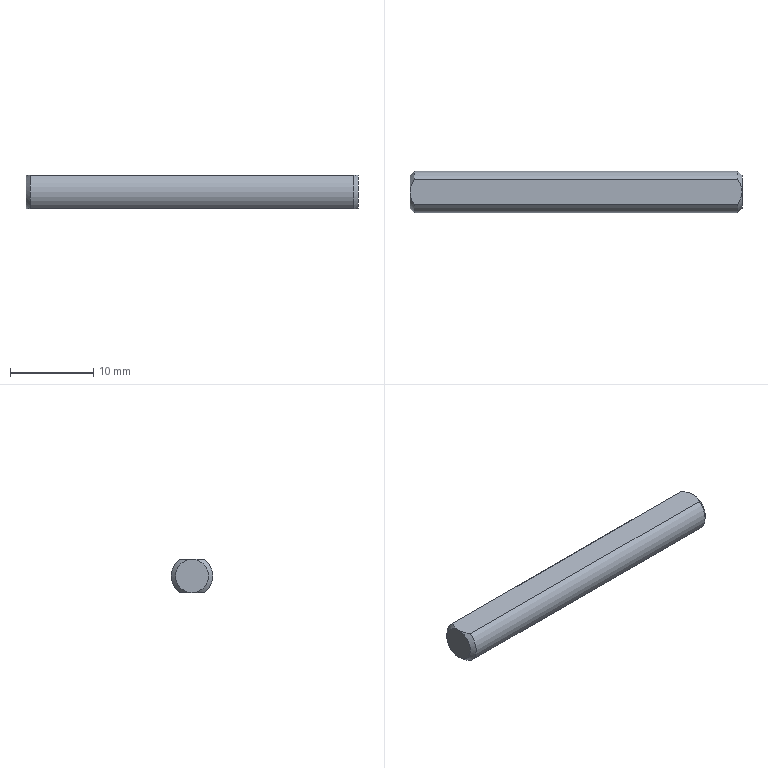Component | SolidWorks | 18ZTJ-NVT-01-003-1 | 1 solid | 10 faces | box 40 x 5 x 4 mm | volume 701 mm3 | cone 4 | plane 4 | cylinder 2 | commonest cylinder face diameters 5 x2 | material #45
build123d program:
from build123d import *

# Parameters (mm, degrees)
SKETCH1_R           = 2.5
BOSS_EXTRUDE1_DEPTH = 40
CHAMFER1_SIZE       = 0.5
CUT_EXTRUDE1_DEPTH  = 41.156


with BuildPart() as part:
    # Sketch1 → Boss-Extrude1 (new body)
    with BuildSketch(Plane(origin=(0, 0, 0), x_dir=(1, 0, 0), z_dir=(0, 1, 0))):
        with Locations(Location((0, 0, 0), (0, 0, 270))):
            Circle(SKETCH1_R)
    extrude(amount=BOSS_EXTRUDE1_DEPTH)

    # Chamfer1
    chamfer1_edges = [part.edges().sort_by_distance(p)[0] for p in [
        (0, 0, -2.5),
        (0, 40, -2.5),
    ]]
    chamfer(chamfer1_edges, length=CHAMFER1_SIZE)

    # Sketch2 → Cut-Extrude1 (cut, through all)
    with BuildSketch(Plane.XZ):
        with BuildLine():
            Line((-1.5, 2), (1.5, 2))
            ThreePointArc((1.5, 2), (0, 2.5), (-1.5, 2))
        make_face()
        with BuildLine():
            Line((-1.5, -2), (1.5, -2))
            ThreePointArc((1.5, -2), (0, -2.5), (-1.5, -2))
        make_face()
    extrude(amount=-CUT_EXTRUDE1_DEPTH, mode=Mode.SUBTRACT)


solid = part.part

# Placed as in the assembly
solid = solid.moved(Location((6.4, -4.53, 111), (0, 0, 90)))
STEP:
#1=COLOUR_RGB('',0.7922,0.8196,0.9333);
#2=FILL_AREA_STYLE_COLOUR('',#1);
#3=FILL_AREA_STYLE('',(#2));
#4=SURFACE_STYLE_FILL_AREA(#3);
#5=SURFACE_SIDE_STYLE('',(#4));
#6=SURFACE_STYLE_USAGE(.BOTH.,#5);
#7=PRESENTATION_STYLE_ASSIGNMENT((#6));
#8=CARTESIAN_POINT('',(-1.303,-0.2374,4.449));
#9=VERTEX_POINT('',#8);
#10=CARTESIAN_POINT('',(-1.303,-0.2374,4.291));
#11=VERTEX_POINT('',#10);
#12=CARTESIAN_POINT('',(-1.303,-0.1783,4.37));
#13=DIRECTION('',(1.,0.,-0.));
#14=DIRECTION('',(0.,-0.,1.));
#15=AXIS2_PLACEMENT_3D('',#12,#13,#14);
#16=CIRCLE('',#15,0.09843);
#17=EDGE_CURVE('',#9,#11,#16,.T.);
#18=ORIENTED_EDGE('',*,*,#17,.T.);
#19=CARTESIAN_POINT('',(0.2323,-0.2374,4.291));
#20=VERTEX_POINT('',#19);
#21=CARTESIAN_POINT('',(-1.323,-0.2374,4.291));
#22=DIRECTION('',(1.,0.,-0.));
#23=VECTOR('',#22,39.37);
#24=LINE('',#21,#23);
#25=EDGE_CURVE('',#11,#20,#24,.T.);
#26=ORIENTED_EDGE('',*,*,#25,.T.);
#27=CARTESIAN_POINT('',(0.2323,-0.2374,4.449));
#28=VERTEX_POINT('',#27);
#29=CARTESIAN_POINT('',(0.2323,-0.1783,4.37));
#30=DIRECTION('',(-1.,-0.,0.));
#31=DIRECTION('',(0.,0.,1.));
#32=AXIS2_PLACEMENT_3D('',#29,#30,#31);
#33=CIRCLE('',#32,0.09843);
#34=EDGE_CURVE('',#20,#28,#33,.T.);
#35=ORIENTED_EDGE('',*,*,#34,.T.);
#36=CARTESIAN_POINT('',(-1.323,-0.2374,4.449));
#37=DIRECTION('',(1.,0.,-0.));
#38=VECTOR('',#37,39.37);
#39=LINE('',#36,#38);
#40=EDGE_CURVE('',#9,#28,#39,.T.);
#41=ORIENTED_EDGE('',*,*,#40,.F.);
#42=EDGE_LOOP('',(#18,#26,#35,#41));
#43=FACE_OUTER_BOUND('',#42,.T.);
#44=CARTESIAN_POINT('',(-1.323,-0.1783,4.37));
#45=DIRECTION('',(1.,0.,-0.));
#46=DIRECTION('',(0.,-0.,-1.));
#47=AXIS2_PLACEMENT_3D('',#44,#45,#46);
#48=CYLINDRICAL_SURFACE('',#47,0.09843);
#49=ADVANCED_FACE('',(#43),#48,.T.);
#50=CARTESIAN_POINT('',(0.2323,-0.1193,4.291));
#51=VERTEX_POINT('',#50);
#52=CARTESIAN_POINT('',(0.252,-0.1783,4.291));
#53=VERTEX_POINT('',#52);
#54=CARTESIAN_POINT('',(0.2323,-0.1193,4.291));
#55=CARTESIAN_POINT('',(0.2377,-0.1283,4.291));
#56=CARTESIAN_POINT('',(0.2425,-0.1376,4.291));
#57=CARTESIAN_POINT('',(0.248,-0.1524,4.291));
#58=CARTESIAN_POINT('',(0.2494,-0.1576,4.291));
#59=CARTESIAN_POINT('',(0.2515,-0.1679,4.291));
#60=CARTESIAN_POINT('',(0.252,-0.1731,4.291));
#61=CARTESIAN_POINT('',(0.252,-0.1783,4.291));
#62=B_SPLINE_CURVE_WITH_KNOTS('',3,(#54,#55,#56,#57,#58,#59,#60,#61),.UNSPECIFIED.,.F.,.F.,(4,2,2,4),(0.005844,0.00664,0.007038,0.007435),.UNSPECIFIED.);
#63=EDGE_CURVE('',#51,#53,#62,.T.);
#64=ORIENTED_EDGE('',*,*,#63,.F.);
#65=CARTESIAN_POINT('',(0.2323,-0.1193,4.449));
#66=VERTEX_POINT('',#65);
#67=CARTESIAN_POINT('',(0.2323,-0.1783,4.37));
#68=DIRECTION('',(-1.,-0.,0.));
#69=DIRECTION('',(0.,0.,1.));
#70=AXIS2_PLACEMENT_3D('',#67,#68,#69);
#71=CIRCLE('',#70,0.09843);
#72=EDGE_CURVE('',#66,#51,#71,.T.);
#73=ORIENTED_EDGE('',*,*,#72,.F.);
#74=CARTESIAN_POINT('',(0.252,-0.1783,4.449));
#75=VERTEX_POINT('',#74);
#76=CARTESIAN_POINT('',(0.252,-0.1783,4.449));
#77=CARTESIAN_POINT('',(0.252,-0.1731,4.449));
#78=CARTESIAN_POINT('',(0.2515,-0.1679,4.449));
#79=CARTESIAN_POINT('',(0.2494,-0.1576,4.449));
#80=CARTESIAN_POINT('',(0.248,-0.1524,4.449));
#81=CARTESIAN_POINT('',(0.2425,-0.1376,4.449));
#82=CARTESIAN_POINT('',(0.2377,-0.1283,4.449));
#83=CARTESIAN_POINT('',(0.2323,-0.1193,4.449));
#84=B_SPLINE_CURVE_WITH_KNOTS('',3,(#76,#77,#78,#79,#80,#81,#82,#83),.UNSPECIFIED.,.F.,.F.,(4,2,2,4),(0.003519,0.003916,0.004313,0.005107),.UNSPECIFIED.);
#85=EDGE_CURVE('',#75,#66,#84,.T.);
#86=ORIENTED_EDGE('',*,*,#85,.F.);
#87=CARTESIAN_POINT('',(0.252,-0.1783,4.37));
#88=DIRECTION('',(1.,0.,-0.));
#89=DIRECTION('',(0.,0.,1.));
#90=AXIS2_PLACEMENT_3D('',#87,#88,#89);
#91=CIRCLE('',#90,0.07874);
#92=EDGE_CURVE('',#53,#75,#91,.T.);
#93=ORIENTED_EDGE('',*,*,#92,.F.);
#94=EDGE_LOOP('',(#64,#73,#86,#93));
#95=FACE_OUTER_BOUND('',#94,.T.);
#96=CARTESIAN_POINT('',(0.2323,-0.1783,4.37));
#97=DIRECTION('',(-1.,-0.,0.));
#98=DIRECTION('',(0.,0.,1.));
#99=AXIS2_PLACEMENT_3D('',#96,#97,#98);
#100=CONICAL_SURFACE('',#99,0.09843,0.7854);
#101=ADVANCED_FACE('',(#95),#100,.T.);
#102=CARTESIAN_POINT('',(-1.323,-0.1783,4.291));
#103=VERTEX_POINT('',#102);
#104=CARTESIAN_POINT('',(-1.303,-0.2374,4.291));
#105=CARTESIAN_POINT('',(-1.309,-0.2284,4.291));
#106=CARTESIAN_POINT('',(-1.313,-0.219,4.291));
#107=CARTESIAN_POINT('',(-1.319,-0.2042,4.291));
#108=CARTESIAN_POINT('',(-1.32,-0.1992,4.291));
#109=CARTESIAN_POINT('',(-1.322,-0.189,4.291));
#110=CARTESIAN_POINT('',(-1.323,-0.1836,4.291));
#111=CARTESIAN_POINT('',(-1.323,-0.1783,4.291));
#112=B_SPLINE_CURVE_WITH_KNOTS('',3,(#104,#105,#106,#107,#108,#109,#110,#111),.UNSPECIFIED.,.F.,.F.,(4,2,2,4),(0.001928,0.002724,0.003122,0.003519),.UNSPECIFIED.);
#113=EDGE_CURVE('',#11,#103,#112,.T.);
#114=ORIENTED_EDGE('',*,*,#113,.F.);
#115=ORIENTED_EDGE('',*,*,#17,.F.);
#116=CARTESIAN_POINT('',(-1.323,-0.1783,4.449));
#117=VERTEX_POINT('',#116);
#118=CARTESIAN_POINT('',(-1.323,-0.1783,4.449));
#119=CARTESIAN_POINT('',(-1.323,-0.1836,4.449));
#120=CARTESIAN_POINT('',(-1.322,-0.189,4.449));
#121=CARTESIAN_POINT('',(-1.32,-0.1992,4.449));
#122=CARTESIAN_POINT('',(-1.319,-0.2042,4.449));
#123=CARTESIAN_POINT('',(-1.313,-0.219,4.449));
#124=CARTESIAN_POINT('',(-1.309,-0.2284,4.449));
#125=CARTESIAN_POINT('',(-1.303,-0.2374,4.449));
#126=B_SPLINE_CURVE_WITH_KNOTS('',3,(#118,#119,#120,#121,#122,#123,#124,#125),.UNSPECIFIED.,.F.,.F.,(4,2,2,4),(0.007435,0.007834,0.008233,0.00903),.UNSPECIFIED.);
#127=EDGE_CURVE('',#117,#9,#126,.T.);
#128=ORIENTED_EDGE('',*,*,#127,.F.);
#129=CARTESIAN_POINT('',(-1.323,-0.1783,4.37));
#130=DIRECTION('',(-1.,-0.,0.));
#131=DIRECTION('',(0.,0.,1.));
#132=AXIS2_PLACEMENT_3D('',#129,#130,#131);
#133=CIRCLE('',#132,0.07874);
#134=EDGE_CURVE('',#103,#117,#133,.T.);
#135=ORIENTED_EDGE('',*,*,#134,.F.);
#136=EDGE_LOOP('',(#114,#115,#128,#135));
#137=FACE_OUTER_BOUND('',#136,.T.);
#138=CARTESIAN_POINT('',(-1.323,-0.1783,4.37));
#139=DIRECTION('',(1.,0.,-0.));
#140=DIRECTION('',(0.,0.,-1.));
#141=AXIS2_PLACEMENT_3D('',#138,#139,#140);
#142=CONICAL_SURFACE('',#141,0.07874,0.7854);
#143=ADVANCED_FACE('',(#137),#142,.T.);
#144=ORIENTED_EDGE('',*,*,#72,.T.);
#145=CARTESIAN_POINT('',(-1.303,-0.1193,4.291));
#146=VERTEX_POINT('',#145);
#147=CARTESIAN_POINT('',(-1.323,-0.1193,4.291));
#148=DIRECTION('',(1.,0.,-0.));
#149=VECTOR('',#148,39.37);
#150=LINE('',#147,#149);
#151=EDGE_CURVE('',#146,#51,#150,.T.);
#152=ORIENTED_EDGE('',*,*,#151,.F.);
#153=CARTESIAN_POINT('',(-1.303,-0.1193,4.449));
#154=VERTEX_POINT('',#153);
#155=CARTESIAN_POINT('',(-1.303,-0.1783,4.37));
#156=DIRECTION('',(1.,0.,-0.));
#157=DIRECTION('',(0.,-0.,1.));
#158=AXIS2_PLACEMENT_3D('',#155,#156,#157);
#159=CIRCLE('',#158,0.09843);
#160=EDGE_CURVE('',#146,#154,#159,.T.);
#161=ORIENTED_EDGE('',*,*,#160,.T.);
#162=CARTESIAN_POINT('',(-1.323,-0.1193,4.449));
#163=DIRECTION('',(1.,0.,-0.));
#164=VECTOR('',#163,39.37);
#165=LINE('',#162,#164);
#166=EDGE_CURVE('',#154,#66,#165,.T.);
#167=ORIENTED_EDGE('',*,*,#166,.T.);
#168=EDGE_LOOP('',(#144,#152,#161,#167));
#169=FACE_OUTER_BOUND('',#168,.T.);
#170=CARTESIAN_POINT('',(-1.323,-0.1783,4.37));
#171=DIRECTION('',(1.,0.,-0.));
#172=DIRECTION('',(0.,-0.,-1.));
#173=AXIS2_PLACEMENT_3D('',#170,#171,#172);
#174=CYLINDRICAL_SURFACE('',#173,0.09843);
#175=ADVANCED_FACE('',(#169),#174,.T.);
#176=CARTESIAN_POINT('',(-1.323,-0.1783,4.37));
#177=DIRECTION('',(-1.,-0.,0.));
#178=DIRECTION('',(0.,0.,1.));
#179=AXIS2_PLACEMENT_3D('',#176,#177,#178);
#180=CIRCLE('',#179,0.07874);
#181=EDGE_CURVE('',#117,#103,#180,.T.);
#182=ORIENTED_EDGE('',*,*,#181,.T.);
#183=ORIENTED_EDGE('',*,*,#134,.T.);
#184=EDGE_LOOP('',(#182,#183));
#185=FACE_OUTER_BOUND('',#184,.T.);
#186=CARTESIAN_POINT('',(-1.323,-0.1783,4.37));
#187=DIRECTION('',(-1.,-0.,0.));
#188=DIRECTION('',(0.,0.,1.));
#189=AXIS2_PLACEMENT_3D('',#186,#187,#188);
#190=PLANE('',#189);
#191=ADVANCED_FACE('',(#185),#190,.T.);
#192=CARTESIAN_POINT('',(0.252,-0.1783,4.37));
#193=DIRECTION('',(1.,0.,-0.));
#194=DIRECTION('',(0.,0.,1.));
#195=AXIS2_PLACEMENT_3D('',#192,#193,#194);
#196=CIRCLE('',#195,0.07874);
#197=EDGE_CURVE('',#75,#53,#196,.T.);
#198=ORIENTED_EDGE('',*,*,#197,.T.);
#199=ORIENTED_EDGE('',*,*,#92,.T.);
#200=EDGE_LOOP('',(#198,#199));
#201=FACE_OUTER_BOUND('',#200,.T.);
#202=CARTESIAN_POINT('',(0.252,-0.1783,4.37));
#203=DIRECTION('',(-1.,-0.,0.));
#204=DIRECTION('',(0.,0.,1.));
#205=AXIS2_PLACEMENT_3D('',#202,#203,#204);
#206=PLANE('',#205);
#207=ADVANCED_FACE('',(#201),#206,.F.);
#208=CARTESIAN_POINT('',(0.252,-0.1783,4.291));
#209=CARTESIAN_POINT('',(0.252,-0.1836,4.291));
#210=CARTESIAN_POINT('',(0.2514,-0.189,4.291));
#211=CARTESIAN_POINT('',(0.2494,-0.1992,4.291));
#212=CARTESIAN_POINT('',(0.248,-0.2042,4.291));
#213=CARTESIAN_POINT('',(0.2426,-0.219,4.291));
#214=CARTESIAN_POINT('',(0.2377,-0.2284,4.291));
#215=CARTESIAN_POINT('',(0.2323,-0.2374,4.291));
#216=B_SPLINE_CURVE_WITH_KNOTS('',3,(#208,#209,#210,#211,#212,#213,#214,#215),.UNSPECIFIED.,.F.,.F.,(4,2,2,4),(0.007435,0.007834,0.008233,0.00903),.UNSPECIFIED.);
#217=EDGE_CURVE('',#53,#20,#216,.T.);
#218=ORIENTED_EDGE('',*,*,#217,.F.);
#219=ORIENTED_EDGE('',*,*,#197,.F.);
#220=CARTESIAN_POINT('',(0.2323,-0.2374,4.449));
#221=CARTESIAN_POINT('',(0.2377,-0.2284,4.449));
#222=CARTESIAN_POINT('',(0.2426,-0.219,4.449));
#223=CARTESIAN_POINT('',(0.248,-0.2042,4.449));
#224=CARTESIAN_POINT('',(0.2494,-0.1992,4.449));
#225=CARTESIAN_POINT('',(0.2514,-0.189,4.449));
#226=CARTESIAN_POINT('',(0.252,-0.1836,4.449));
#227=CARTESIAN_POINT('',(0.252,-0.1783,4.449));
#228=B_SPLINE_CURVE_WITH_KNOTS('',3,(#220,#221,#222,#223,#224,#225,#226,#227),.UNSPECIFIED.,.F.,.F.,(4,2,2,4),(0.001928,0.002724,0.003122,0.003519),.UNSPECIFIED.);
#229=EDGE_CURVE('',#28,#75,#228,.T.);
#230=ORIENTED_EDGE('',*,*,#229,.F.);
#231=ORIENTED_EDGE('',*,*,#34,.F.);
#232=EDGE_LOOP('',(#218,#219,#230,#231));
#233=FACE_OUTER_BOUND('',#232,.T.);
#234=CARTESIAN_POINT('',(0.2323,-0.1783,4.37));
#235=DIRECTION('',(-1.,-0.,0.));
#236=DIRECTION('',(0.,0.,1.));
#237=AXIS2_PLACEMENT_3D('',#234,#235,#236);
#238=CONICAL_SURFACE('',#237,0.09843,0.7854);
#239=ADVANCED_FACE('',(#233),#238,.T.);
#240=CARTESIAN_POINT('',(-1.323,-0.1783,4.291));
#241=CARTESIAN_POINT('',(-1.323,-0.1731,4.291));
#242=CARTESIAN_POINT('',(-1.322,-0.1679,4.291));
#243=CARTESIAN_POINT('',(-1.32,-0.1576,4.291));
#244=CARTESIAN_POINT('',(-1.319,-0.1524,4.291));
#245=CARTESIAN_POINT('',(-1.313,-0.1376,4.291));
#246=CARTESIAN_POINT('',(-1.309,-0.1283,4.291));
#247=CARTESIAN_POINT('',(-1.303,-0.1193,4.291));
#248=B_SPLINE_CURVE_WITH_KNOTS('',3,(#240,#241,#242,#243,#244,#245,#246,#247),.UNSPECIFIED.,.F.,.F.,(4,2,2,4),(0.003519,0.003916,0.004313,0.005107),.UNSPECIFIED.);
#249=EDGE_CURVE('',#103,#146,#248,.T.);
#250=ORIENTED_EDGE('',*,*,#249,.F.);
#251=ORIENTED_EDGE('',*,*,#181,.F.);
#252=CARTESIAN_POINT('',(-1.303,-0.1193,4.449));
#253=CARTESIAN_POINT('',(-1.309,-0.1283,4.449));
#254=CARTESIAN_POINT('',(-1.313,-0.1376,4.449));
#255=CARTESIAN_POINT('',(-1.319,-0.1524,4.449));
#256=CARTESIAN_POINT('',(-1.32,-0.1576,4.449));
#257=CARTESIAN_POINT('',(-1.322,-0.1679,4.449));
#258=CARTESIAN_POINT('',(-1.323,-0.1731,4.449));
#259=CARTESIAN_POINT('',(-1.323,-0.1783,4.449));
#260=B_SPLINE_CURVE_WITH_KNOTS('',3,(#252,#253,#254,#255,#256,#257,#258,#259),.UNSPECIFIED.,.F.,.F.,(4,2,2,4),(0.005844,0.00664,0.007038,0.007435),.UNSPECIFIED.);
#261=EDGE_CURVE('',#154,#117,#260,.T.);
#262=ORIENTED_EDGE('',*,*,#261,.F.);
#263=ORIENTED_EDGE('',*,*,#160,.F.);
#264=EDGE_LOOP('',(#250,#251,#262,#263));
#265=FACE_OUTER_BOUND('',#264,.T.);
#266=CARTESIAN_POINT('',(-1.323,-0.1783,4.37));
#267=DIRECTION('',(1.,0.,-0.));
#268=DIRECTION('',(0.,0.,-1.));
#269=AXIS2_PLACEMENT_3D('',#266,#267,#268);
#270=CONICAL_SURFACE('',#269,0.07874,0.7854);
#271=ADVANCED_FACE('',(#265),#270,.T.);
#272=ORIENTED_EDGE('',*,*,#229,.T.);
#273=ORIENTED_EDGE('',*,*,#85,.T.);
#274=ORIENTED_EDGE('',*,*,#166,.F.);
#275=ORIENTED_EDGE('',*,*,#261,.T.);
#276=ORIENTED_EDGE('',*,*,#127,.T.);
#277=ORIENTED_EDGE('',*,*,#40,.T.);
#278=EDGE_LOOP('',(#272,#273,#274,#275,#276,#277));
#279=FACE_OUTER_BOUND('',#278,.T.);
#280=CARTESIAN_POINT('',(-1.323,-0.2374,4.449));
#281=DIRECTION('',(-0.,-0.,-1.));
#282=DIRECTION('',(-0.,-1.,0.));
#283=AXIS2_PLACEMENT_3D('',#280,#281,#282);
#284=PLANE('',#283);
#285=ADVANCED_FACE('',(#279),#284,.F.);
#286=ORIENTED_EDGE('',*,*,#63,.T.);
#287=ORIENTED_EDGE('',*,*,#217,.T.);
#288=ORIENTED_EDGE('',*,*,#25,.F.);
#289=ORIENTED_EDGE('',*,*,#113,.T.);
#290=ORIENTED_EDGE('',*,*,#249,.T.);
#291=ORIENTED_EDGE('',*,*,#151,.T.);
#292=EDGE_LOOP('',(#286,#287,#288,#289,#290,#291));
#293=FACE_OUTER_BOUND('',#292,.T.);
#294=CARTESIAN_POINT('',(-1.323,-0.2374,4.291));
#295=DIRECTION('',(0.,0.,1.));
#296=DIRECTION('',(0.,1.,-0.));
#297=AXIS2_PLACEMENT_3D('',#294,#295,#296);
#298=PLANE('',#297);
#299=ADVANCED_FACE('',(#293),#298,.F.);
#300=CLOSED_SHELL('',(#49,#101,#143,#175,#191,#207,#239,#271,#285,#299));
#301=MANIFOLD_SOLID_BREP('',#300);
#302=STYLED_ITEM('',(#7),#301);
#303=PRESENTATION_LAYER_ASSIGNMENT('','',(#302));
#304=CARTESIAN_POINT('',(0.,0.,0.));
#305=DIRECTION('',(0.,0.,1.));
#306=DIRECTION('',(1.,0.,0.));
#307=AXIS2_PLACEMENT_3D('',#304,#305,#306);
#308=(LENGTH_UNIT()NAMED_UNIT(*)SI_UNIT($,.METRE.));
#309=LENGTH_MEASURE_WITH_UNIT(LENGTH_MEASURE(0.0254),#308);
#310=DIMENSIONAL_EXPONENTS(1.,0.,0.,0.,0.,0.,0.);
#311=(CONVERSION_BASED_UNIT('',#309)LENGTH_UNIT()NAMED_UNIT(#310));
#312=UNCERTAINTY_MEASURE_WITH_UNIT(LENGTH_MEASURE(0.00001),#311,'','');
#313=(NAMED_UNIT(*)PLANE_ANGLE_UNIT()SI_UNIT($,.RADIAN.));
#314=(NAMED_UNIT(*)SI_UNIT($,.STERADIAN.)SOLID_ANGLE_UNIT());
#315=(GEOMETRIC_REPRESENTATION_CONTEXT(3)GLOBAL_UNCERTAINTY_ASSIGNED_CONTEXT((#312))GLOBAL_UNIT_ASSIGNED_CONTEXT((#311,#313,#314))REPRESENTATION_CONTEXT('',''));
#316=ADVANCED_BREP_SHAPE_REPRESENTATION('',(#301,#307),#315);
#317=(LENGTH_UNIT()NAMED_UNIT(*)SI_UNIT($,.METRE.));
#318=LENGTH_MEASURE_WITH_UNIT(LENGTH_MEASURE(0.0254),#317);
#319=DIMENSIONAL_EXPONENTS(1.,0.,0.,0.,0.,0.,0.);
#320=(CONVERSION_BASED_UNIT('',#318)LENGTH_UNIT()NAMED_UNIT(#319));
#321=UNCERTAINTY_MEASURE_WITH_UNIT(LENGTH_MEASURE(0.00001),#320,'','');
#322=(NAMED_UNIT(*)PLANE_ANGLE_UNIT()SI_UNIT($,.RADIAN.));
#323=(NAMED_UNIT(*)SI_UNIT($,.STERADIAN.)SOLID_ANGLE_UNIT());
#324=(GEOMETRIC_REPRESENTATION_CONTEXT(3)GLOBAL_UNCERTAINTY_ASSIGNED_CONTEXT((#321))GLOBAL_UNIT_ASSIGNED_CONTEXT((#320,#322,#323))REPRESENTATION_CONTEXT('',''));
#325=MECHANICAL_DESIGN_GEOMETRIC_PRESENTATION_REPRESENTATION('',(#302),#324);